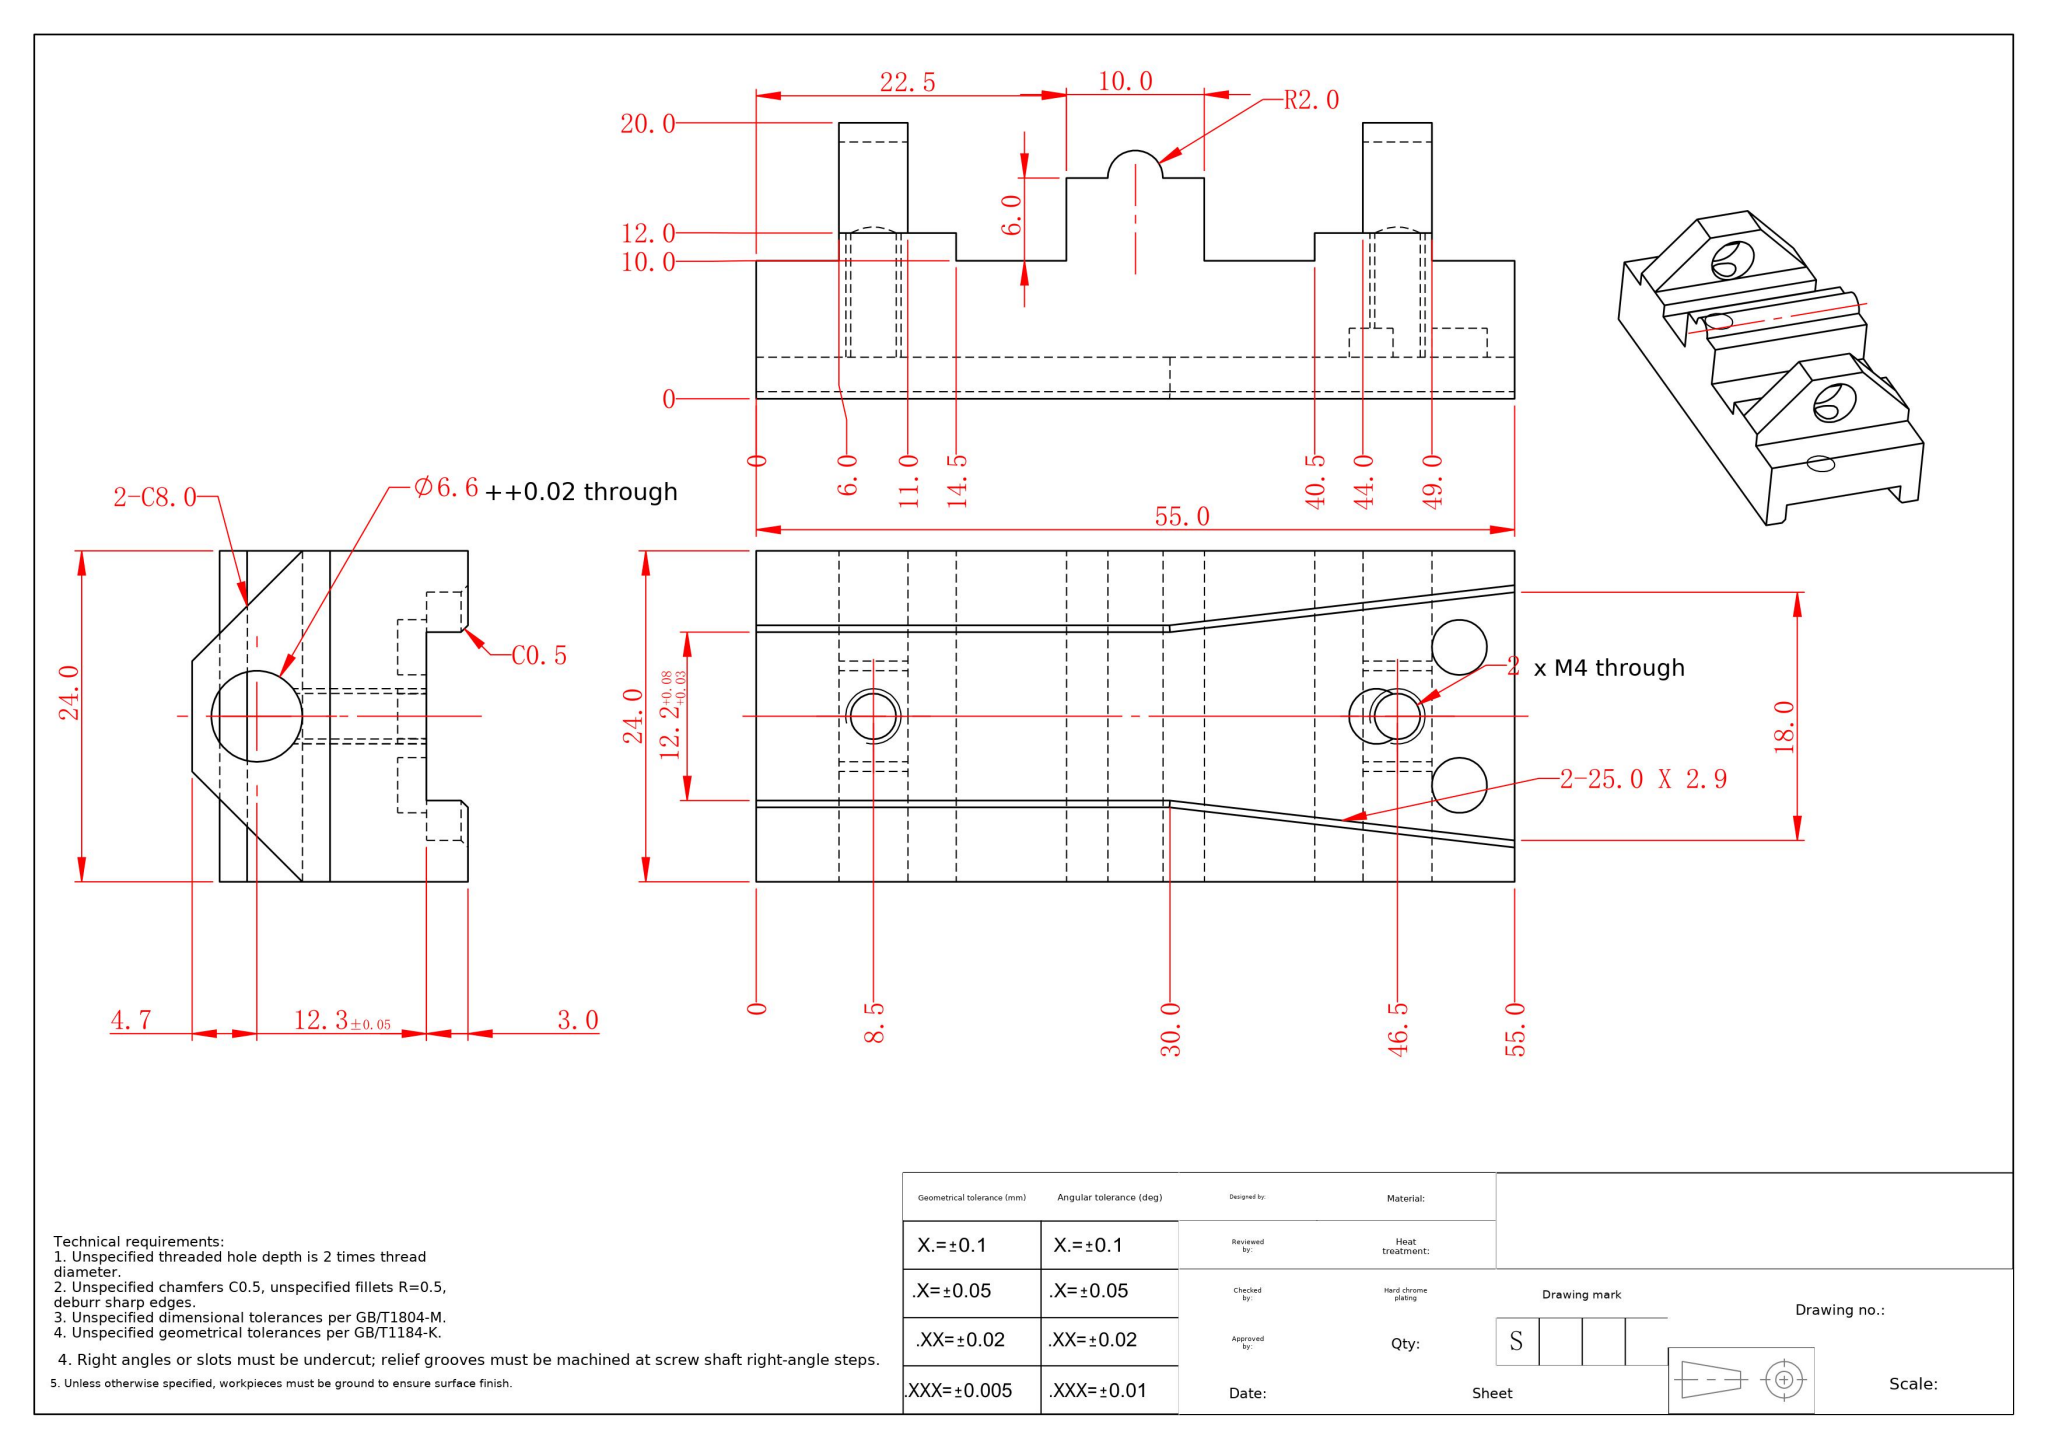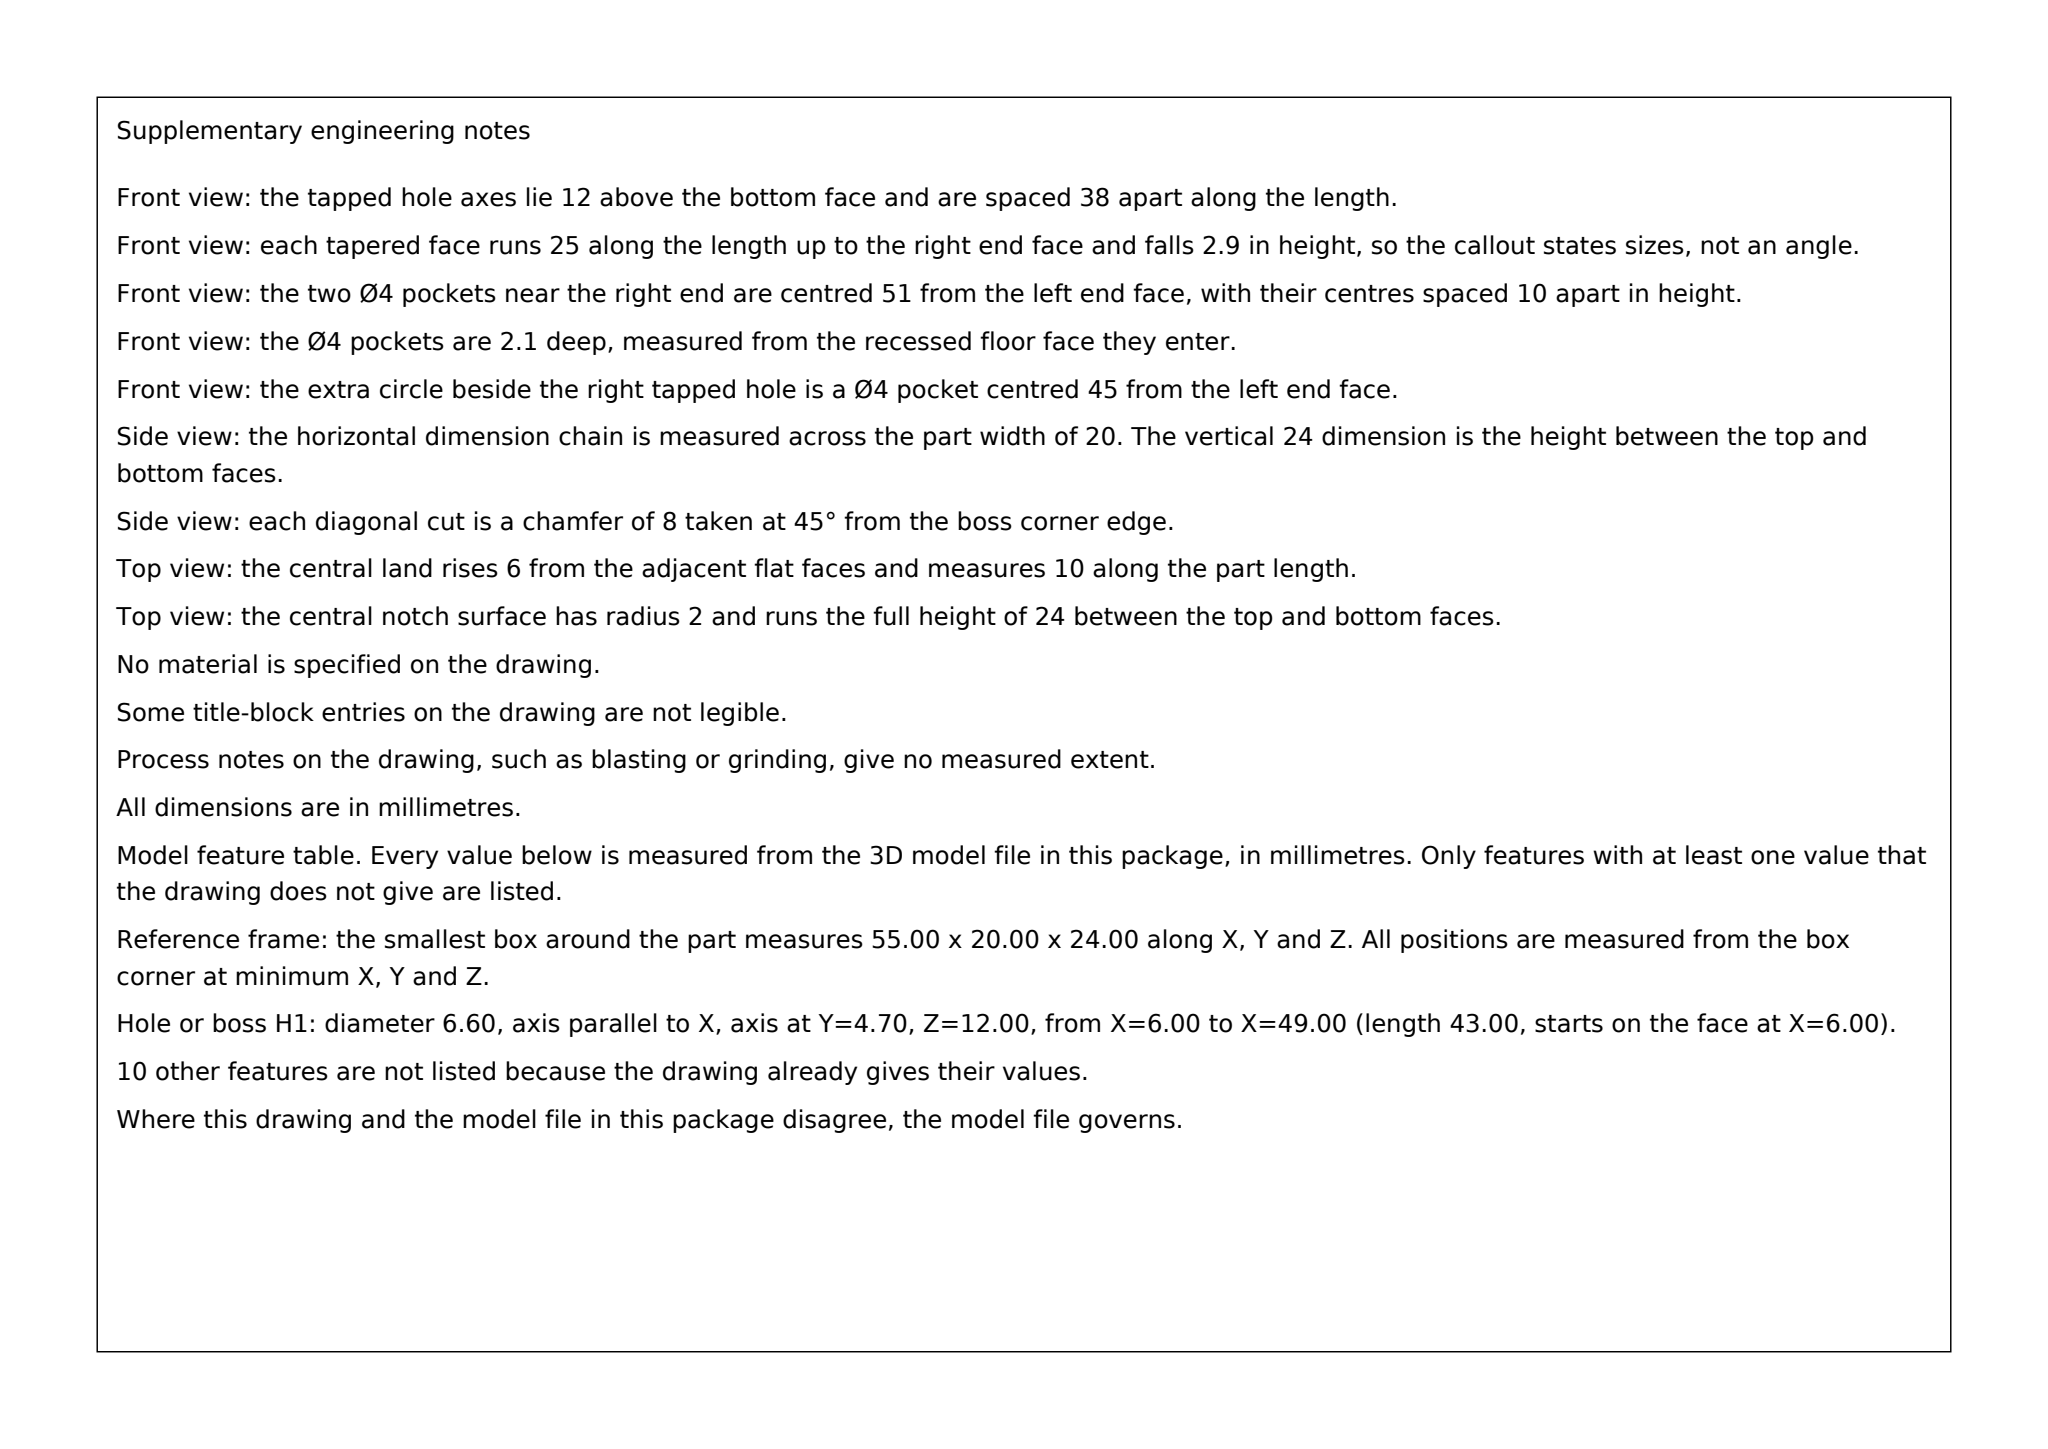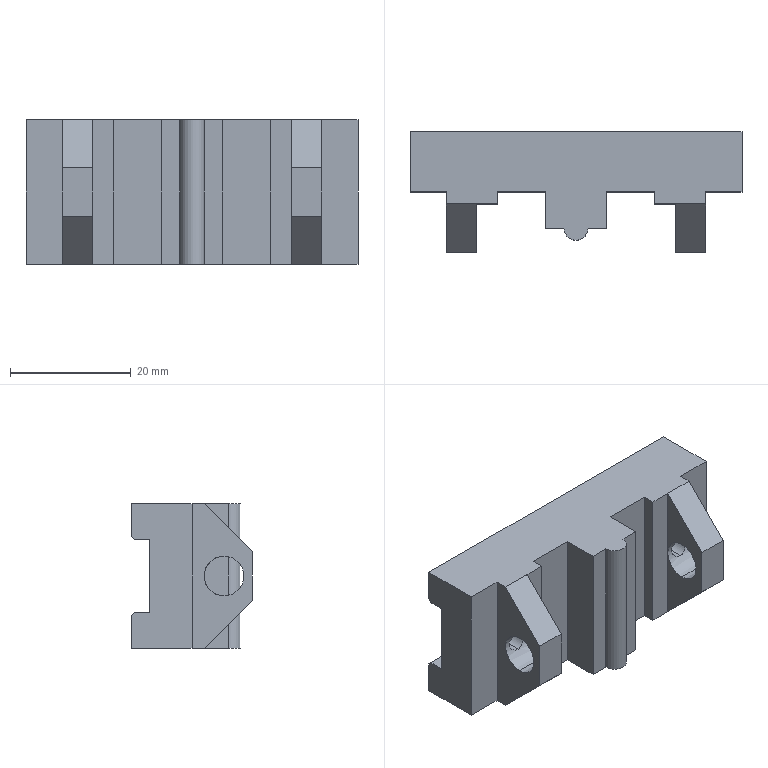Part | SolidWorks | mm | 1 solid | 56 faces | box 55 x 20 x 24 mm | volume 14076 mm3 | plane 40 | cylinder 16 | commonest cylinder face diameters 4 x8 3.3 x4 6.6 x4
Drawing notes:
2X SIDE TAPER RELIEF X30.0-X55.0, 2.9 DP EA SIDE, 18.2 W AT END | from the solid: x planes 30.0 & 55.0 (25.0 lg); bbox z 24.0 less 2.9 per side = 18.2
2X M4 THRU: X8.5 & X46.5 FROM LH END, Z12.0 ON CL | from the solid: cyl dia3.3 axis y at (8.5,z12.0) and (46.5,z12.0), len 9.44
3X Ø4.0 DP 2.1: X45.0 Z12.0; X51.0 Z7.0 & Z17.0 FROM LH END/BTM | from the solid: cyl dia4.0 axis y at (x45.0,z12.0), (x51.0,z7.0), (x51.0,z17.0), len 2.1
Ø4.0 THRU 24 WIDTH, AT X27.5, 4.0 UP FROM BASE (FRONT VIEW) | from the solid: cylinder [4.0,'z',[27.5,4.0,null],24.0,1]; bbox z=24.0, y origin at base
2X SIDE TAPER RELIEF 2.9 DP: Y8.0 TO Y10.0 (2.0 HIGH) FROM BASE | from the solid: y-planes at 8.0 and 10.0 bound the relief faces; base at y=0, so relief spans 8.0-10.0 above bottom face
BOTTOM UNDERCUT: 12.2 WIDE x 4.0 DP, FULL LEN X0 TO X55.0 | from the solid: z-planes 5.9/18.1 (=12.2 wide, centred on z12.0); y-planes 0 and 4.0; runs x0 to x55 (bbox length)
12.2 +0.08/+0.03 SLOT: 4.0 DP FROM BOTTOM FACE (Y0 TO Y4.0) | from the solid: slot walls z=5.9/18.1 (12.2), roof at y=4.0 above bottom face y=0
3X Ø4.0 DP 2.1 FROM Y14.9 FLAT, 5.1 BELOW TOP FACE Y20.0 | from the solid: 3X dia4.0 y-axis cyl len 2.1 at (45.0,z12.0),(51.0,z7.0),(51.0,z17.0); y-planes at 14.9 (3) and top 20.0
build123d program:
from build123d import *

# Parameters (mm, degrees)
SKETCH1_W              = 55
SKETCH1_H              = 20
BOSS_EXTRUDE1_DEPTH    = 24
CUT_EXTRUDE1_REACH     = 39.845
SKETCH2_W              = 33
SKETCH2_H              = 8
SKETCH2_W_2            = 6
SKETCH2_H_2            = 10
SKETCH4_R              = 3.3
CUT_EXTRUDE2_DEPTH     = 56.471
CUT_EXTRUDE3_REACH     = 39.845
SKETCH5_W              = 26
SKETCH5_H              = 2
CUT_EXTRUDE4_DEPTH     = 3
CHAMFER1_SIZE          = 8
M4_TAPPED_HOLE2_REACH  = 42.265
M4_TAPPED_HOLE2_BORE_R = 1.65
CHAMFER2_SIZE          = 0.5
SKETCH11_R             = 2
CUT_EXTRUDE5_DEPTH     = 2.1
BOSS_EXTRUDE2_DEPTH    = 24


with BuildPart() as part:
    # Sketch1 → Boss-Extrude1 (new body)
    with BuildSketch(Plane.XY):
        Rectangle(SKETCH1_W, SKETCH1_H)
    extrude(amount=BOSS_EXTRUDE1_DEPTH)

    # Sketch2 → Cut-Extrude1 (cut, up to next)
    with BuildSketch(Plane.XY.offset(24), mode=Mode.PRIVATE) as cut_extrude1_sk1:
        with Locations((0, -6)):
            Rectangle(SKETCH2_W, SKETCH2_H)
    cut_extrude1_tool1 = extrude(cut_extrude1_sk1.sketch, amount=-CUT_EXTRUDE1_REACH, mode=Mode.PRIVATE) & part.part
    # Sketch2 → Cut-Extrude1 (cut, up to next)
    with BuildSketch(Plane.XY.offset(24), mode=Mode.PRIVATE) as cut_extrude1_sk2:
        with Locations((-24.5, -5)):
            Rectangle(SKETCH2_W_2, SKETCH2_H_2)
    cut_extrude1_tool2 = extrude(cut_extrude1_sk2.sketch, amount=-CUT_EXTRUDE1_REACH, mode=Mode.PRIVATE) & part.part
    # Sketch2 → Cut-Extrude1 (cut, up to next)
    with BuildSketch(Plane.XY.offset(24), mode=Mode.PRIVATE) as cut_extrude1_sk3:
        with Locations((24.5, -5)):
            Rectangle(SKETCH2_W_2, SKETCH2_H_2)
    cut_extrude1_tool3 = extrude(cut_extrude1_sk3.sketch, amount=-CUT_EXTRUDE1_REACH, mode=Mode.PRIVATE) & part.part
    add(cut_extrude1_tool1.solids().sort_by_distance((0, -6, 24))[0], mode=Mode.SUBTRACT)
    add(cut_extrude1_tool2.solids().sort_by_distance((-24.5, -5, 24))[0], mode=Mode.SUBTRACT)
    add(cut_extrude1_tool3.solids().sort_by_distance((24.5, -5, 24))[0], mode=Mode.SUBTRACT)

    # Sketch4 → Cut-Extrude2 (cut, through all)
    with BuildSketch(Plane.ZY.offset(21.5)):
        with Locations((12, -5.3)):
            Circle(SKETCH4_R)
    extrude(amount=-CUT_EXTRUDE2_DEPTH, mode=Mode.SUBTRACT)

    # Sketch5 → Cut-Extrude3 (cut, up to next)
    with BuildSketch(Plane.XY.offset(24), mode=Mode.PRIVATE) as cut_extrude3_sk1:
        with Locations((0, -1)):
            Rectangle(SKETCH5_W, SKETCH5_H)
    cut_extrude3_tool1 = extrude(cut_extrude3_sk1.sketch, amount=-CUT_EXTRUDE3_REACH, mode=Mode.PRIVATE) & part.part
    add(cut_extrude3_tool1.solids().sort_by_distance((0, -1, 24))[0], mode=Mode.SUBTRACT)

    # Sketch6 → Cut-Extrude4 (cut)
    with BuildSketch(Plane(origin=(0, 10, 0), x_dir=(1, 0, 0), z_dir=(0, 1, 0))):
        Polygon((-27.5, -18.1), (2.5, -18.1), (27.5, -21), (27.5, -3), (2.5, -5.9), (-27.5, -5.9), align=None)
    extrude(amount=-CUT_EXTRUDE4_DEPTH, mode=Mode.SUBTRACT)

    # Chamfer1
    chamfer1_edges = [part.edges().sort_by_distance(p)[0] for p in [
        (19, -10, 24),
        (19, -10, 0),
        (-19, -10, 0),
        (-19, -10, 24),
    ]]
    chamfer(chamfer1_edges, length=CHAMFER1_SIZE)

    # M4 Tapped Hole2 bore → M4 Tapped Hole2 (cut, up to next)
    with BuildSketch(Plane(origin=(0, 7, 0), x_dir=(1, 0, 0), z_dir=(0, 1, 0)), mode=Mode.PRIVATE) as m4_tapped_hole2_sk1:
        with Locations((-19, -12)):
            Circle(M4_TAPPED_HOLE2_BORE_R)
    m4_tapped_hole2_tool1 = extrude(m4_tapped_hole2_sk1.sketch, amount=-M4_TAPPED_HOLE2_REACH, mode=Mode.PRIVATE) & part.part
    # M4 Tapped Hole2 bore → M4 Tapped Hole2 (cut, up to next)
    with BuildSketch(Plane(origin=(0, 7, 0), x_dir=(1, 0, 0), z_dir=(0, 1, 0)), mode=Mode.PRIVATE) as m4_tapped_hole2_sk2:
        with Locations((19, -12)):
            Circle(M4_TAPPED_HOLE2_BORE_R)
    m4_tapped_hole2_tool2 = extrude(m4_tapped_hole2_sk2.sketch, amount=-M4_TAPPED_HOLE2_REACH, mode=Mode.PRIVATE) & part.part
    add(m4_tapped_hole2_tool1.solids().sort_by_distance((-19, 7, 12))[0], mode=Mode.SUBTRACT)
    add(m4_tapped_hole2_tool2.solids().sort_by_distance((19, 7, 12))[0], mode=Mode.SUBTRACT)

    # Chamfer2
    chamfer2_edges = [part.edges().sort_by_distance(p)[0] for p in [
        (-12.5, 10, 18.1),
        (15, 10, 19.55),
        (15, 10, 4.45),
        (-12.5, 10, 5.9),
    ]]
    chamfer(chamfer2_edges, length=CHAMFER2_SIZE)

    # Sketch11 → Cut-Extrude5 (cut)
    with BuildSketch(Plane(origin=(0, 7, 0), x_dir=(1, 0, 0), z_dir=(0, 1, 0))):
        with Locations((17.5, -12)):
            Circle(SKETCH11_R)
        with Locations(Location((23.5, -7, 0), (0, 0, 270))):
            Circle(SKETCH11_R)
        with Locations(Location((23.5, -17, 0), (0, 0, 90))):
            Circle(SKETCH11_R)
    extrude(amount=-CUT_EXTRUDE5_DEPTH, mode=Mode.SUBTRACT)

    # Sketch12 → Boss-Extrude2 (add)
    with BuildSketch(Plane(origin=(0, 0, 0), x_dir=(-1, 0, 0), z_dir=(0, 0, -1))):
        with BuildLine():
            Line((-5, 0), (5, 0))
            Line((5, 0), (5, -6))
            Line((5, -6), (2, -6))
            ThreePointArc((2, -6), (0, -8), (-2, -6))
            Line((-2, -6), (-5, -6))
            Line((-5, -6), (-5, 0))
        make_face()
    extrude(amount=-BOSS_EXTRUDE2_DEPTH)


solid = part.part